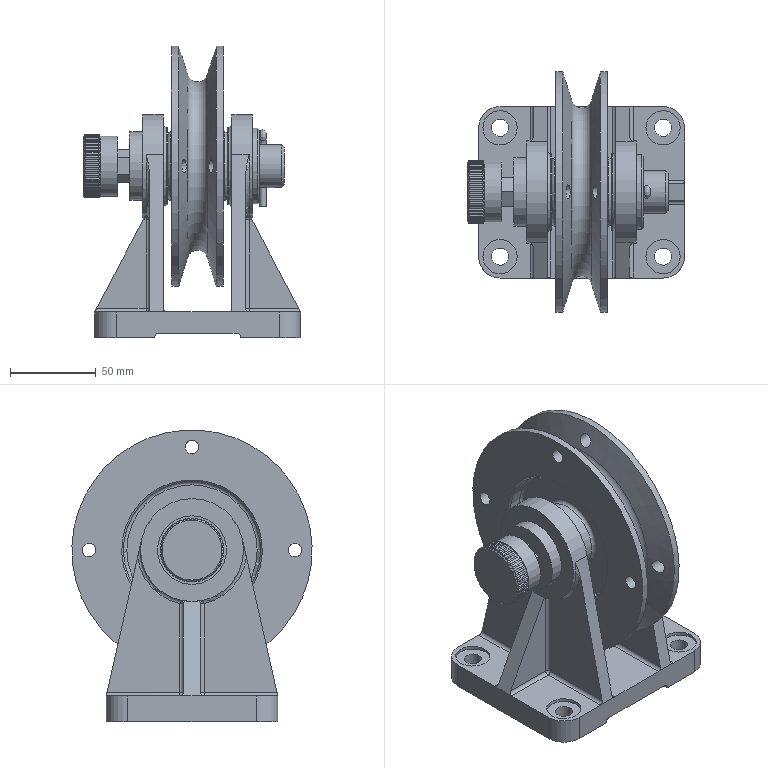Assembly | NX | mm | 7 component files | 7 solids | 298 faces | box 126.5 x 140 x 170 mm | volume 639938 mm3 | cylinder 175 | plane 80 | cone 19 | torus 15 | sphere 8 | spline 1 | commonest cylinder face diameters 37 x50 1 x50 4 x23 25 x9 8 x8 10 x5 20 x4 40 x3
Bill of materials:
GB-T91-2000,3.7x32 | 1 |  | Split Pin, GB-T 91-2000,3.7x32
unnamed part 1 | 1 |  | Stepped, hollow body of revolution. It has a large round flange that tapers through a conical shoulder into a hexagonal prism section, followed by a smaller cylindrical spigot with a chamfered end. A central bore runs through the full length.
unnamed part 2 | 1 |  | Cylindrical cap or cup shape. One end is closed by a flat face and has a band of axial ribs or flutes around the outside. The other section is a plain cylindrical sleeve with an open end and a thin wall.
unnamed part 3 | 1 |  | Headed cylindrical pin. A flat round head sits at one end of a long plain shank that has a chamfered tip. The shank has two small radial holes along its length.
unnamed part 4 | 1 |  | Clevis-style bracket. A rectangular base plate with rounded corners carries two parallel upright lugs. Each lug tapers upward to a rounded top with a circular eye hole and a raised ring boss. The lugs are spaced apart with a gap between them.
unnamed part 5 | 1 |  | Grooved wheel or sheave. The rim has a deep, round-bottomed groove. The central hub has a through bore, and hub bosses stick out slightly from both side faces. Each face has a recessed annular area, and four small holes are evenly spaced near the outer edge.
unnamed part 6 | 1 |  | Flat annular ring, washer-like in shape. It is a thin disc with a large central hole and a small chamfer on one outer edge.
Mates:
1. fix | 1_bracket 1 component
2. touch align | 5_pulley 1 face | 1_bracket 1 face
3. center | 5_pulley 1 face | 5_pulley 1 face | 1_bracket 1 face | 1_bracket 1 face
4. touch align | 2_mandrel 1 face | 1_bracket 1 face
5. touch align | 2_mandrel 1 face | 1_bracket 1 face
6. touch align | 4_flat_washer 1 face | 2_mandrel 1 face
7. touch align | 4_flat_washer 1 face | 1_bracket 1 face
8. touch align | 3_cotter_pin 1 face | 2_mandrel 1 face
9. touch align | 6_oil_cup_body 1 face | 2_mandrel 1 face
10. touch align | 6_oil_cup_body 1 face | 2_mandrel 1 face
11. touch align | 7_oil_cup_body 1 face | 6_oil_cup_body 1 face
12. touch align | 7_oil_cup_body 1 face | 6_oil_cup_body 1 face